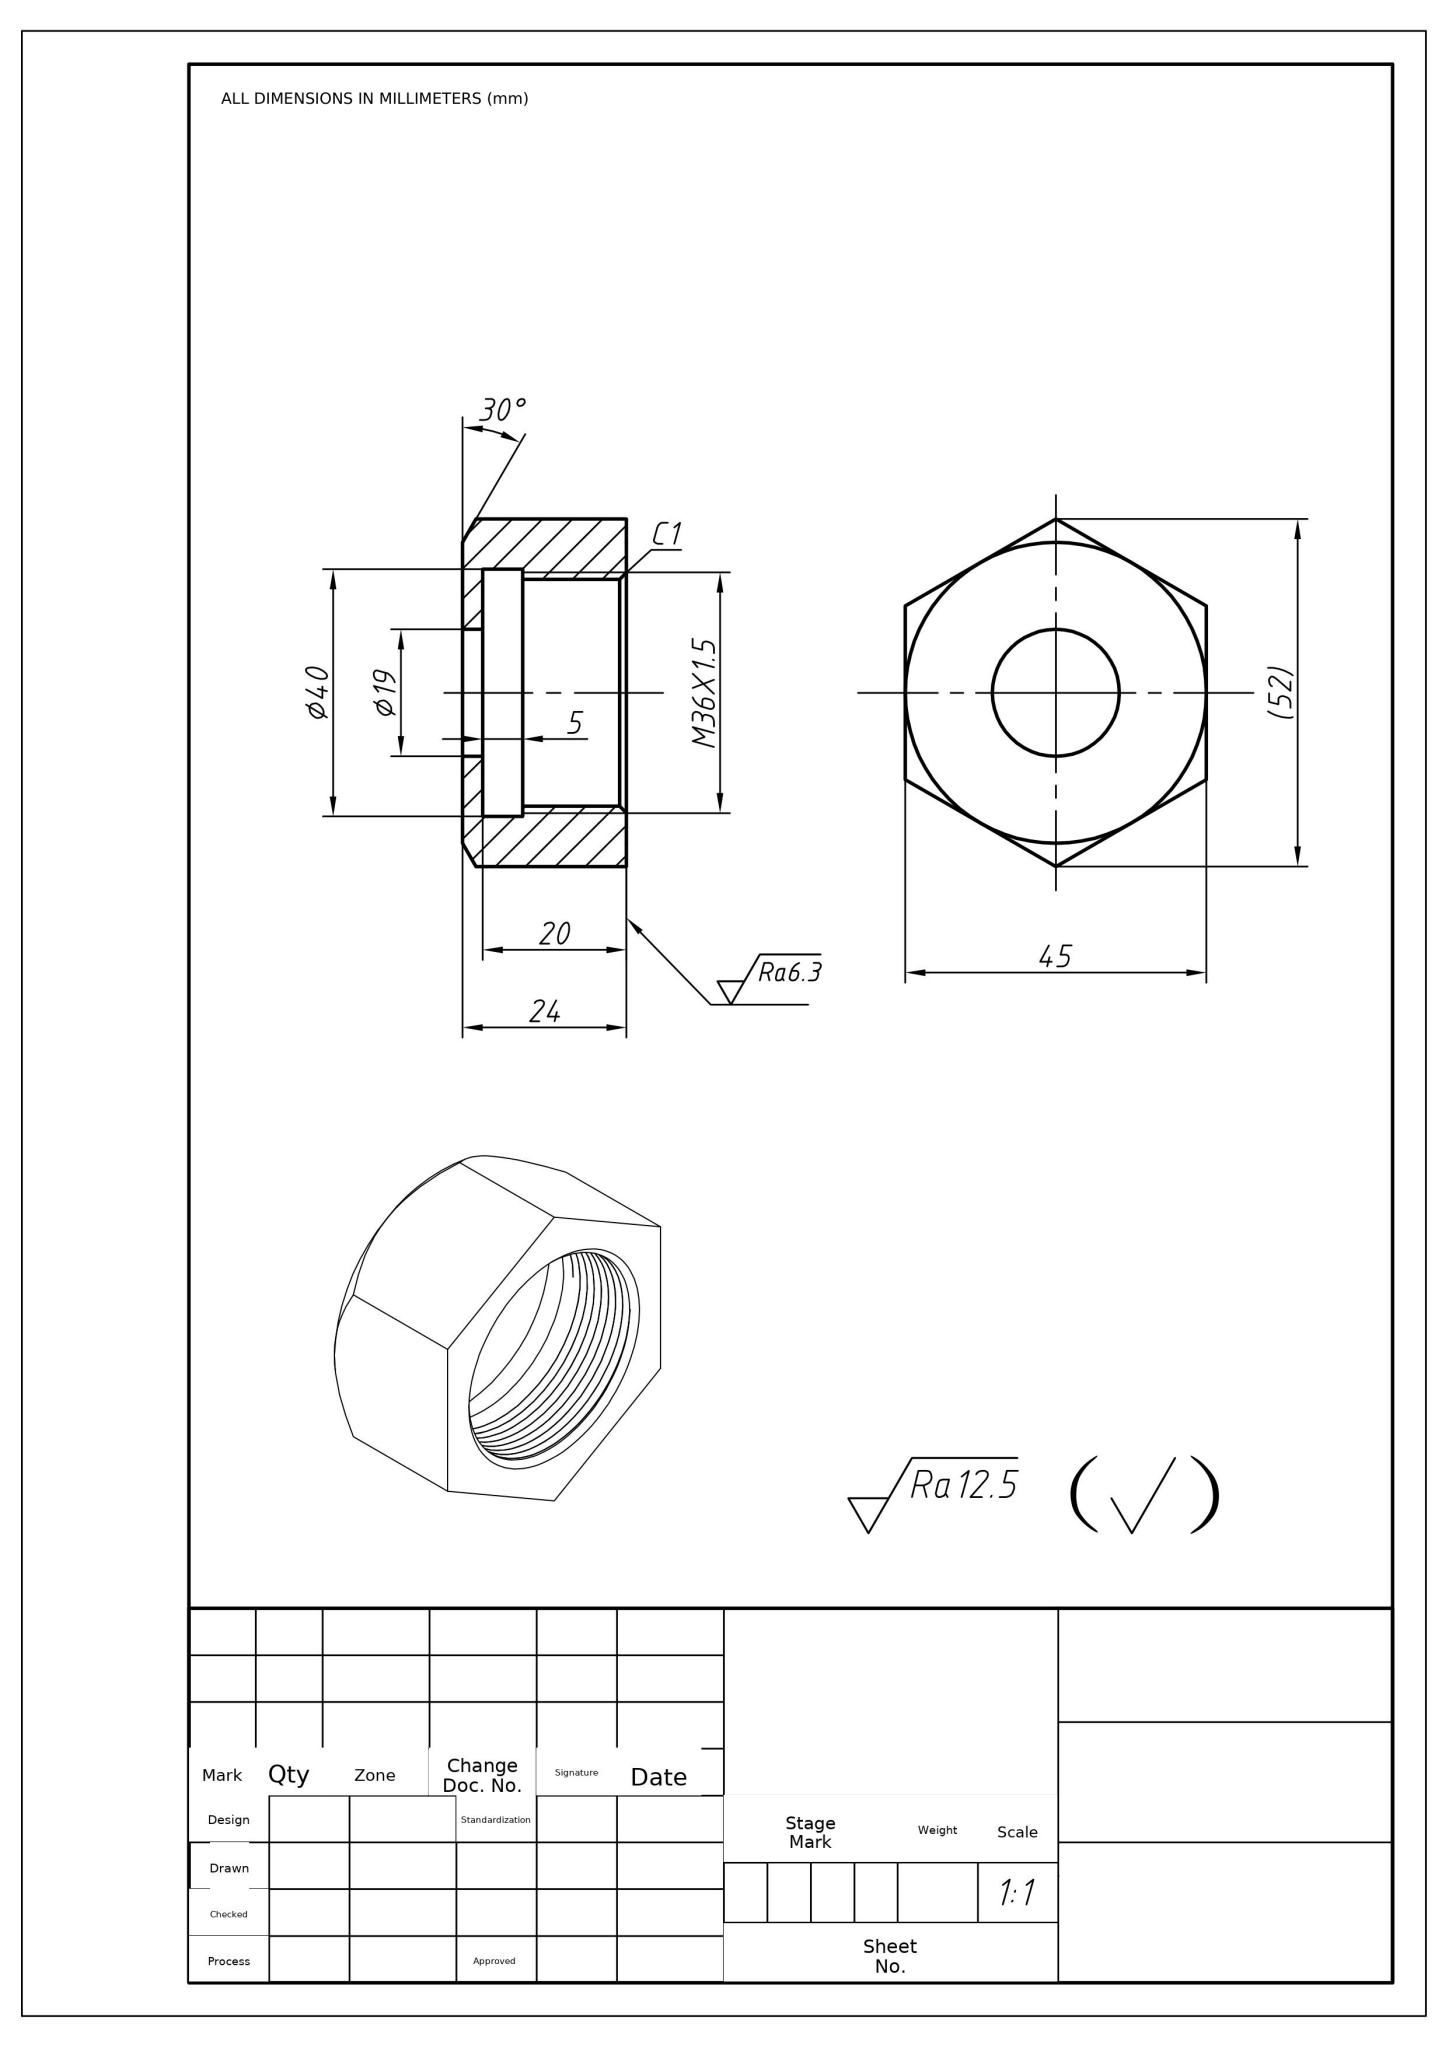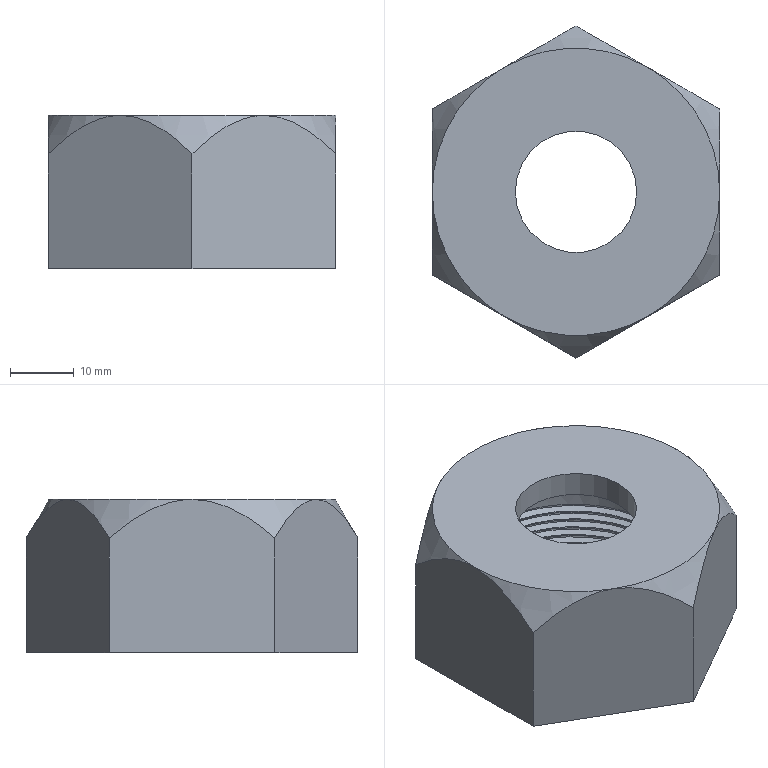Part | NX | mm | 1 solid | 32 faces | box 45 x 51.96 x 24 mm | volume 19753 mm3 | cylinder 12 | plane 11 | cone 7 | spline 2 | commonest cylinder face diameters 34.376 x9 40 x1 19 x1 36 x1